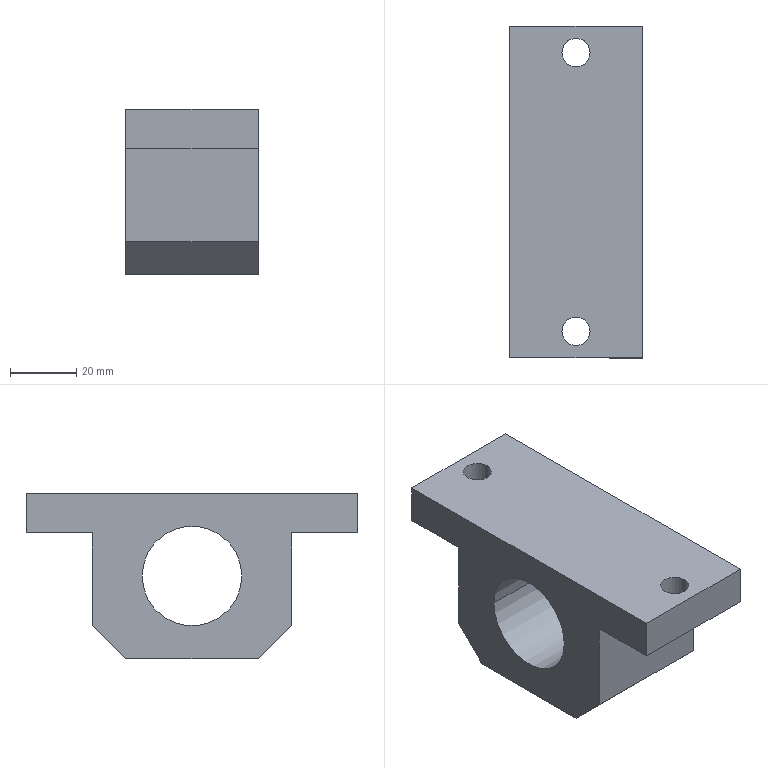Component | SolidWorks | AxisSeat-1 | 1 solid | 20 faces | box 40 x 100 x 50 mm | volume 105366 mm3 | plane 12 | cylinder 8 | commonest cylinder face diameters 8.5 x4 5 x2 30 x2
build123d program:
from build123d import *

# Parameters (mm, degrees)
SKETCH1_R              = 15
BOSS_EXTRUDE1_DEPTH    = 40
SKETCH2_R              = 4.25
CUT_EXTRUDE1_DEPTH     = 82.24
CHAMFER1_SIZE          = 10
M6_TAPPED_HOLE1_REACH  = 83.24
M6_TAPPED_HOLE1_BORE_R = 2.5


with BuildPart() as part:
    # Sketch1 → Boss-Extrude1 (new body)
    with BuildSketch(Plane.XY):
        Polygon((-50, 0), (-50, 12), (-30, 12), (-30, 50), (30, 50), (30, 12), (50, 12), (50, 0), align=None)
        with Locations((0, 25)):
            Circle(SKETCH1_R, mode=Mode.SUBTRACT)
    extrude(amount=BOSS_EXTRUDE1_DEPTH)

    # Sketch2 → Cut-Extrude1 (cut, through all)
    with BuildSketch(Plane.XZ):
        with Locations(Location((-42, 20, 0), (0, 0, 270))):
            Circle(SKETCH2_R)
        with Locations(Location((42, 20, 0), (0, 0, 270))):
            Circle(SKETCH2_R)
    extrude(amount=-CUT_EXTRUDE1_DEPTH, mode=Mode.SUBTRACT)

    # Chamfer1
    chamfer1_edges = [part.edges().sort_by_distance(p)[0] for p in [
        (-30, 50, 20),
        (30, 50, 20),
    ]]
    chamfer(chamfer1_edges, length=CHAMFER1_SIZE)

    # M6 Tapped Hole1 bore → M6 Tapped Hole1 (cut, up to next)
    with BuildSketch(Plane(origin=(0, 50, 0), x_dir=(1, 0, 0), z_dir=(0, 1, 0)), mode=Mode.PRIVATE) as m6_tapped_hole1_sk1:
        with Locations((0, -20)):
            Circle(M6_TAPPED_HOLE1_BORE_R)
    m6_tapped_hole1_tool1 = extrude(m6_tapped_hole1_sk1.sketch, amount=-M6_TAPPED_HOLE1_REACH, mode=Mode.PRIVATE) & part.part
    add(m6_tapped_hole1_tool1.solids().sort_by_distance((0, 50, 20))[0], mode=Mode.SUBTRACT)


solid = part.part

# Placed as in the assembly
solid = solid.moved(Location((894.468, -62.684, 1336.399), (-90, 90, 0)))
STEP:
#1=COLOUR_RGB('',0.7922,0.8196,0.9333);
#2=FILL_AREA_STYLE_COLOUR('',#1);
#3=FILL_AREA_STYLE('',(#2));
#4=SURFACE_STYLE_FILL_AREA(#3);
#5=SURFACE_SIDE_STYLE('',(#4));
#6=SURFACE_STYLE_USAGE(.BOTH.,#5);
#7=PRESENTATION_STYLE_ASSIGNMENT((#6));
#8=CARTESIAN_POINT('',(35.904,-2.468,51.039));
#9=VERTEX_POINT('',#8);
#10=CARTESIAN_POINT('',(36.101,-2.468,51.039));
#11=VERTEX_POINT('',#10);
#12=CARTESIAN_POINT('',(35.904,-2.468,51.039));
#13=CARTESIAN_POINT('',(35.904,-2.474,51.039));
#14=CARTESIAN_POINT('',(35.905,-2.481,51.039));
#15=CARTESIAN_POINT('',(35.907,-2.493,51.04));
#16=CARTESIAN_POINT('',(35.909,-2.5,51.04));
#17=CARTESIAN_POINT('',(35.914,-2.512,51.041));
#18=CARTESIAN_POINT('',(35.917,-2.517,51.041));
#19=CARTESIAN_POINT('',(35.924,-2.528,51.042));
#20=CARTESIAN_POINT('',(35.929,-2.533,51.043));
#21=CARTESIAN_POINT('',(35.942,-2.547,51.045));
#22=CARTESIAN_POINT('',(35.953,-2.554,51.046));
#23=CARTESIAN_POINT('',(35.971,-2.561,51.047));
#24=CARTESIAN_POINT('',(35.977,-2.563,51.047));
#25=CARTESIAN_POINT('',(35.99,-2.566,51.047));
#26=CARTESIAN_POINT('',(35.996,-2.566,51.048));
#27=CARTESIAN_POINT('',(36.009,-2.566,51.048));
#28=CARTESIAN_POINT('',(36.016,-2.566,51.047));
#29=CARTESIAN_POINT('',(36.028,-2.563,51.047));
#30=CARTESIAN_POINT('',(36.034,-2.561,51.047));
#31=CARTESIAN_POINT('',(36.046,-2.556,51.046));
#32=CARTESIAN_POINT('',(36.052,-2.553,51.046));
#33=CARTESIAN_POINT('',(36.063,-2.546,51.045));
#34=CARTESIAN_POINT('',(36.068,-2.542,51.044));
#35=CARTESIAN_POINT('',(36.077,-2.533,51.043));
#36=CARTESIAN_POINT('',(36.081,-2.528,51.042));
#37=CARTESIAN_POINT('',(36.088,-2.517,51.041));
#38=CARTESIAN_POINT('',(36.091,-2.512,51.041));
#39=CARTESIAN_POINT('',(36.096,-2.5,51.04));
#40=CARTESIAN_POINT('',(36.098,-2.493,51.04));
#41=CARTESIAN_POINT('',(36.1,-2.481,51.039));
#42=CARTESIAN_POINT('',(36.101,-2.474,51.039));
#43=CARTESIAN_POINT('',(36.101,-2.468,51.039));
#44=B_SPLINE_CURVE_WITH_KNOTS('',3,(#12,#13,#14,#15,#16,#17,#18,#19,#20,#21,#22,#23,#24,#25,#26,#27,#28,#29,#30,#31,#32,#33,#34,#35,#36,#37,#38,#39,#40,#41,#42,#43),.UNSPECIFIED.,.F.,.F.,(4,2,2,2,2,2,2,2,2,2,2,2,2,2,2,4),(0.,0.0004894,0.0009787,0.001468,0.001957,0.002936,0.003426,0.003915,0.004404,0.004894,0.005383,0.005872,0.006362,0.006851,0.00734,0.00783),.UNSPECIFIED.);
#45=EDGE_CURVE('',#9,#11,#44,.T.);
#46=ORIENTED_EDGE('',*,*,#45,.T.);
#47=CARTESIAN_POINT('',(36.101,-2.468,50.646));
#48=VERTEX_POINT('',#47);
#49=CARTESIAN_POINT('',(36.101,-2.468,50.646));
#50=DIRECTION('',(0.,0.,-1.));
#51=VECTOR('',#50,39.37);
#52=LINE('',#49,#51);
#53=EDGE_CURVE('',#11,#48,#52,.T.);
#54=ORIENTED_EDGE('',*,*,#53,.T.);
#55=CARTESIAN_POINT('',(35.904,-2.468,50.646));
#56=VERTEX_POINT('',#55);
#57=CARTESIAN_POINT('',(36.003,-2.468,50.646));
#58=DIRECTION('',(0.,0.,-1.));
#59=DIRECTION('',(-1.,0.,0.));
#60=AXIS2_PLACEMENT_3D('',#57,#58,#59);
#61=CIRCLE('',#60,0.09843);
#62=EDGE_CURVE('',#48,#56,#61,.T.);
#63=ORIENTED_EDGE('',*,*,#62,.T.);
#64=CARTESIAN_POINT('',(35.904,-2.468,50.646));
#65=DIRECTION('',(0.,0.,-1.));
#66=VECTOR('',#65,39.37);
#67=LINE('',#64,#66);
#68=EDGE_CURVE('',#9,#56,#67,.T.);
#69=ORIENTED_EDGE('',*,*,#68,.F.);
#70=EDGE_LOOP('',(#46,#54,#63,#69));
#71=FACE_OUTER_BOUND('',#70,.T.);
#72=CARTESIAN_POINT('',(36.003,-2.468,50.646));
#73=DIRECTION('',(0.,0.,-1.));
#74=DIRECTION('',(-1.,0.,0.));
#75=AXIS2_PLACEMENT_3D('',#72,#73,#74);
#76=CYLINDRICAL_SURFACE('',#75,0.09843);
#77=ADVANCED_FACE('',(#71),#76,.F.);
#78=CARTESIAN_POINT('',(35.835,-0.8143,52.142));
#79=VERTEX_POINT('',#78);
#80=CARTESIAN_POINT('',(36.17,-0.8143,52.142));
#81=VERTEX_POINT('',#80);
#82=CARTESIAN_POINT('',(36.003,-0.8143,52.142));
#83=DIRECTION('',(-0.,0.,1.));
#84=DIRECTION('',(0.,1.,0.));
#85=AXIS2_PLACEMENT_3D('',#82,#83,#84);
#86=CIRCLE('',#85,0.1673);
#87=EDGE_CURVE('',#79,#81,#86,.T.);
#88=ORIENTED_EDGE('',*,*,#87,.F.);
#89=CARTESIAN_POINT('',(35.835,-0.8143,52.614));
#90=VERTEX_POINT('',#89);
#91=CARTESIAN_POINT('',(35.835,-0.8143,50.646));
#92=DIRECTION('',(-0.,-0.,1.));
#93=VECTOR('',#92,39.37);
#94=LINE('',#91,#93);
#95=EDGE_CURVE('',#79,#90,#94,.T.);
#96=ORIENTED_EDGE('',*,*,#95,.T.);
#97=CARTESIAN_POINT('',(36.17,-0.8143,52.614));
#98=VERTEX_POINT('',#97);
#99=CARTESIAN_POINT('',(36.003,-0.8143,52.614));
#100=DIRECTION('',(-0.,-0.,1.));
#101=DIRECTION('',(1.,0.,0.));
#102=AXIS2_PLACEMENT_3D('',#99,#100,#101);
#103=CIRCLE('',#102,0.1673);
#104=EDGE_CURVE('',#90,#98,#103,.T.);
#105=ORIENTED_EDGE('',*,*,#104,.T.);
#106=CARTESIAN_POINT('',(36.17,-0.8143,50.646));
#107=DIRECTION('',(-0.,-0.,1.));
#108=VECTOR('',#107,39.37);
#109=LINE('',#106,#108);
#110=EDGE_CURVE('',#81,#98,#109,.T.);
#111=ORIENTED_EDGE('',*,*,#110,.F.);
#112=EDGE_LOOP('',(#88,#96,#105,#111));
#113=FACE_OUTER_BOUND('',#112,.T.);
#114=CARTESIAN_POINT('',(36.003,-0.8143,50.646));
#115=DIRECTION('',(-0.,-0.,1.));
#116=DIRECTION('',(1.,0.,0.));
#117=AXIS2_PLACEMENT_3D('',#114,#115,#116);
#118=CYLINDRICAL_SURFACE('',#117,0.1673);
#119=ADVANCED_FACE('',(#113),#118,.F.);
#120=CARTESIAN_POINT('',(35.835,-4.121,52.142));
#121=VERTEX_POINT('',#120);
#122=CARTESIAN_POINT('',(36.17,-4.121,52.142));
#123=VERTEX_POINT('',#122);
#124=CARTESIAN_POINT('',(36.003,-4.121,52.142));
#125=DIRECTION('',(-0.,-0.,1.));
#126=DIRECTION('',(1.,0.,0.));
#127=AXIS2_PLACEMENT_3D('',#124,#125,#126);
#128=CIRCLE('',#127,0.1673);
#129=EDGE_CURVE('',#121,#123,#128,.T.);
#130=ORIENTED_EDGE('',*,*,#129,.F.);
#131=CARTESIAN_POINT('',(35.835,-4.121,52.614));
#132=VERTEX_POINT('',#131);
#133=CARTESIAN_POINT('',(35.835,-4.121,50.646));
#134=DIRECTION('',(-0.,-0.,1.));
#135=VECTOR('',#134,39.37);
#136=LINE('',#133,#135);
#137=EDGE_CURVE('',#121,#132,#136,.T.);
#138=ORIENTED_EDGE('',*,*,#137,.T.);
#139=CARTESIAN_POINT('',(36.17,-4.121,52.614));
#140=VERTEX_POINT('',#139);
#141=CARTESIAN_POINT('',(36.003,-4.121,52.614));
#142=DIRECTION('',(-0.,-0.,1.));
#143=DIRECTION('',(1.,0.,0.));
#144=AXIS2_PLACEMENT_3D('',#141,#142,#143);
#145=CIRCLE('',#144,0.1673);
#146=EDGE_CURVE('',#132,#140,#145,.T.);
#147=ORIENTED_EDGE('',*,*,#146,.T.);
#148=CARTESIAN_POINT('',(36.17,-4.121,50.646));
#149=DIRECTION('',(-0.,-0.,1.));
#150=VECTOR('',#149,39.37);
#151=LINE('',#148,#150);
#152=EDGE_CURVE('',#123,#140,#151,.T.);
#153=ORIENTED_EDGE('',*,*,#152,.F.);
#154=EDGE_LOOP('',(#130,#138,#147,#153));
#155=FACE_OUTER_BOUND('',#154,.T.);
#156=CARTESIAN_POINT('',(36.003,-4.121,50.646));
#157=DIRECTION('',(-0.,-0.,1.));
#158=DIRECTION('',(1.,0.,0.));
#159=AXIS2_PLACEMENT_3D('',#156,#157,#158);
#160=CYLINDRICAL_SURFACE('',#159,0.1673);
#161=ADVANCED_FACE('',(#155),#160,.F.);
#162=CARTESIAN_POINT('',(35.215,-3.058,51.63));
#163=VERTEX_POINT('',#162);
#164=CARTESIAN_POINT('',(35.215,-1.877,51.63));
#165=VERTEX_POINT('',#164);
#166=CARTESIAN_POINT('',(35.215,-2.468,51.63));
#167=DIRECTION('',(-1.,0.,-0.));
#168=DIRECTION('',(0.,1.,0.));
#169=AXIS2_PLACEMENT_3D('',#166,#167,#168);
#170=CIRCLE('',#169,0.5906);
#171=EDGE_CURVE('',#163,#165,#170,.T.);
#172=ORIENTED_EDGE('',*,*,#171,.T.);
#173=CARTESIAN_POINT('',(36.79,-1.877,51.63));
#174=VERTEX_POINT('',#173);
#175=CARTESIAN_POINT('',(35.215,-1.877,51.63));
#176=DIRECTION('',(1.,-0.,0.));
#177=VECTOR('',#176,39.37);
#178=LINE('',#175,#177);
#179=EDGE_CURVE('',#165,#174,#178,.T.);
#180=ORIENTED_EDGE('',*,*,#179,.T.);
#181=CARTESIAN_POINT('',(36.79,-3.058,51.63));
#182=VERTEX_POINT('',#181);
#183=CARTESIAN_POINT('',(36.79,-2.468,51.63));
#184=DIRECTION('',(-1.,0.,-0.));
#185=DIRECTION('',(0.,1.,0.));
#186=AXIS2_PLACEMENT_3D('',#183,#184,#185);
#187=CIRCLE('',#186,0.5906);
#188=EDGE_CURVE('',#182,#174,#187,.T.);
#189=ORIENTED_EDGE('',*,*,#188,.F.);
#190=CARTESIAN_POINT('',(35.215,-3.058,51.63));
#191=DIRECTION('',(1.,-0.,0.));
#192=VECTOR('',#191,39.37);
#193=LINE('',#190,#192);
#194=EDGE_CURVE('',#163,#182,#193,.T.);
#195=ORIENTED_EDGE('',*,*,#194,.F.);
#196=EDGE_LOOP('',(#172,#180,#189,#195));
#197=FACE_OUTER_BOUND('',#196,.T.);
#198=CARTESIAN_POINT('',(35.215,-2.468,51.63));
#199=DIRECTION('',(1.,-0.,0.));
#200=DIRECTION('',(0.,-1.,0.));
#201=AXIS2_PLACEMENT_3D('',#198,#199,#200);
#202=CYLINDRICAL_SURFACE('',#201,0.5906);
#203=ADVANCED_FACE('',(#197),#202,.F.);
#204=CARTESIAN_POINT('',(35.215,-1.287,52.142));
#205=VERTEX_POINT('',#204);
#206=CARTESIAN_POINT('',(35.215,-1.287,51.039));
#207=VERTEX_POINT('',#206);
#208=CARTESIAN_POINT('',(35.215,-1.287,50.646));
#209=DIRECTION('',(0.,-0.,-1.));
#210=VECTOR('',#209,39.37);
#211=LINE('',#208,#210);
#212=EDGE_CURVE('',#205,#207,#211,.T.);
#213=ORIENTED_EDGE('',*,*,#212,.T.);
#214=CARTESIAN_POINT('',(35.215,-1.68,50.646));
#215=VERTEX_POINT('',#214);
#216=CARTESIAN_POINT('',(35.215,-1.09,51.236));
#217=DIRECTION('',(0.,-0.7071,-0.7071));
#218=VECTOR('',#217,39.37);
#219=LINE('',#216,#218);
#220=EDGE_CURVE('',#207,#215,#219,.T.);
#221=ORIENTED_EDGE('',*,*,#220,.T.);
#222=CARTESIAN_POINT('',(35.215,-3.255,50.646));
#223=VERTEX_POINT('',#222);
#224=CARTESIAN_POINT('',(35.215,-3.649,50.646));
#225=DIRECTION('',(-0.,-1.,-0.));
#226=VECTOR('',#225,39.37);
#227=LINE('',#224,#226);
#228=EDGE_CURVE('',#215,#223,#227,.T.);
#229=ORIENTED_EDGE('',*,*,#228,.T.);
#230=CARTESIAN_POINT('',(35.215,-3.649,51.039));
#231=VERTEX_POINT('',#230);
#232=CARTESIAN_POINT('',(35.215,-3.846,51.236));
#233=DIRECTION('',(-0.,-0.7071,0.7071));
#234=VECTOR('',#233,39.37);
#235=LINE('',#232,#234);
#236=EDGE_CURVE('',#223,#231,#235,.T.);
#237=ORIENTED_EDGE('',*,*,#236,.T.);
#238=CARTESIAN_POINT('',(35.215,-3.649,52.142));
#239=VERTEX_POINT('',#238);
#240=CARTESIAN_POINT('',(35.215,-3.649,50.646));
#241=DIRECTION('',(-0.,-0.,1.));
#242=VECTOR('',#241,39.37);
#243=LINE('',#240,#242);
#244=EDGE_CURVE('',#231,#239,#243,.T.);
#245=ORIENTED_EDGE('',*,*,#244,.T.);
#246=CARTESIAN_POINT('',(35.215,-4.436,52.142));
#247=VERTEX_POINT('',#246);
#248=CARTESIAN_POINT('',(35.215,-4.436,52.142));
#249=DIRECTION('',(-0.,-1.,-0.));
#250=VECTOR('',#249,39.37);
#251=LINE('',#248,#250);
#252=EDGE_CURVE('',#239,#247,#251,.T.);
#253=ORIENTED_EDGE('',*,*,#252,.T.);
#254=CARTESIAN_POINT('',(35.215,-4.436,52.614));
#255=VERTEX_POINT('',#254);
#256=CARTESIAN_POINT('',(35.215,-4.436,52.614));
#257=DIRECTION('',(-0.,-0.,1.));
#258=VECTOR('',#257,39.37);
#259=LINE('',#256,#258);
#260=EDGE_CURVE('',#247,#255,#259,.T.);
#261=ORIENTED_EDGE('',*,*,#260,.T.);
#262=CARTESIAN_POINT('',(35.215,-0.4994,52.614));
#263=VERTEX_POINT('',#262);
#264=CARTESIAN_POINT('',(35.215,-4.436,52.614));
#265=DIRECTION('',(0.,1.,0.));
#266=VECTOR('',#265,39.37);
#267=LINE('',#264,#266);
#268=EDGE_CURVE('',#255,#263,#267,.T.);
#269=ORIENTED_EDGE('',*,*,#268,.T.);
#270=CARTESIAN_POINT('',(35.215,-0.4994,52.142));
#271=VERTEX_POINT('',#270);
#272=CARTESIAN_POINT('',(35.215,-0.4994,52.614));
#273=DIRECTION('',(0.,0.,-1.));
#274=VECTOR('',#273,39.37);
#275=LINE('',#272,#274);
#276=EDGE_CURVE('',#263,#271,#275,.T.);
#277=ORIENTED_EDGE('',*,*,#276,.T.);
#278=CARTESIAN_POINT('',(35.215,-0.4994,52.142));
#279=DIRECTION('',(-0.,-1.,0.));
#280=VECTOR('',#279,39.37);
#281=LINE('',#278,#280);
#282=EDGE_CURVE('',#271,#205,#281,.T.);
#283=ORIENTED_EDGE('',*,*,#282,.T.);
#284=EDGE_LOOP('',(#213,#221,#229,#237,#245,#253,#261,#269,#277,#283));
#285=FACE_OUTER_BOUND('',#284,.T.);
#286=ORIENTED_EDGE('',*,*,#171,.F.);
#287=CARTESIAN_POINT('',(35.215,-2.468,51.63));
#288=DIRECTION('',(-1.,0.,-0.));
#289=DIRECTION('',(0.,1.,0.));
#290=AXIS2_PLACEMENT_3D('',#287,#288,#289);
#291=CIRCLE('',#290,0.5906);
#292=EDGE_CURVE('',#165,#163,#291,.T.);
#293=ORIENTED_EDGE('',*,*,#292,.F.);
#294=EDGE_LOOP('',(#286,#293));
#295=FACE_BOUND('',#294,.T.);
#296=CARTESIAN_POINT('',(35.215,-2.468,52.614));
#297=DIRECTION('',(-1.,0.,-0.));
#298=DIRECTION('',(0.,1.,0.));
#299=AXIS2_PLACEMENT_3D('',#296,#297,#298);
#300=PLANE('',#299);
#301=ADVANCED_FACE('',(#285,#295),#300,.T.);
#302=CARTESIAN_POINT('',(36.79,-1.68,50.646));
#303=VERTEX_POINT('',#302);
#304=CARTESIAN_POINT('',(36.79,-3.255,50.646));
#305=VERTEX_POINT('',#304);
#306=CARTESIAN_POINT('',(36.79,-3.649,50.646));
#307=DIRECTION('',(-0.,-1.,-0.));
#308=VECTOR('',#307,39.37);
#309=LINE('',#306,#308);
#310=EDGE_CURVE('',#303,#305,#309,.T.);
#311=ORIENTED_EDGE('',*,*,#310,.F.);
#312=CARTESIAN_POINT('',(36.79,-1.287,51.039));
#313=VERTEX_POINT('',#312);
#314=CARTESIAN_POINT('',(36.79,-1.68,50.646));
#315=DIRECTION('',(-0.,0.7071,0.7071));
#316=VECTOR('',#315,39.37);
#317=LINE('',#314,#316);
#318=EDGE_CURVE('',#303,#313,#317,.T.);
#319=ORIENTED_EDGE('',*,*,#318,.T.);
#320=CARTESIAN_POINT('',(36.79,-1.287,52.142));
#321=VERTEX_POINT('',#320);
#322=CARTESIAN_POINT('',(36.79,-1.287,50.646));
#323=DIRECTION('',(0.,-0.,-1.));
#324=VECTOR('',#323,39.37);
#325=LINE('',#322,#324);
#326=EDGE_CURVE('',#321,#313,#325,.T.);
#327=ORIENTED_EDGE('',*,*,#326,.F.);
#328=CARTESIAN_POINT('',(36.79,-0.4994,52.142));
#329=VERTEX_POINT('',#328);
#330=CARTESIAN_POINT('',(36.79,-0.4994,52.142));
#331=DIRECTION('',(-0.,-1.,0.));
#332=VECTOR('',#331,39.37);
#333=LINE('',#330,#332);
#334=EDGE_CURVE('',#329,#321,#333,.T.);
#335=ORIENTED_EDGE('',*,*,#334,.F.);
#336=CARTESIAN_POINT('',(36.79,-0.4994,52.614));
#337=VERTEX_POINT('',#336);
#338=CARTESIAN_POINT('',(36.79,-0.4994,52.614));
#339=DIRECTION('',(0.,0.,-1.));
#340=VECTOR('',#339,39.37);
#341=LINE('',#338,#340);
#342=EDGE_CURVE('',#337,#329,#341,.T.);
#343=ORIENTED_EDGE('',*,*,#342,.F.);
#344=CARTESIAN_POINT('',(36.79,-4.436,52.614));
#345=VERTEX_POINT('',#344);
#346=CARTESIAN_POINT('',(36.79,-4.436,52.614));
#347=DIRECTION('',(0.,1.,0.));
#348=VECTOR('',#347,39.37);
#349=LINE('',#346,#348);
#350=EDGE_CURVE('',#345,#337,#349,.T.);
#351=ORIENTED_EDGE('',*,*,#350,.F.);
#352=CARTESIAN_POINT('',(36.79,-4.436,52.142));
#353=VERTEX_POINT('',#352);
#354=CARTESIAN_POINT('',(36.79,-4.436,52.614));
#355=DIRECTION('',(-0.,-0.,1.));
#356=VECTOR('',#355,39.37);
#357=LINE('',#354,#356);
#358=EDGE_CURVE('',#353,#345,#357,.T.);
#359=ORIENTED_EDGE('',*,*,#358,.F.);
#360=CARTESIAN_POINT('',(36.79,-3.649,52.142));
#361=VERTEX_POINT('',#360);
#362=CARTESIAN_POINT('',(36.79,-4.436,52.142));
#363=DIRECTION('',(-0.,-1.,-0.));
#364=VECTOR('',#363,39.37);
#365=LINE('',#362,#364);
#366=EDGE_CURVE('',#361,#353,#365,.T.);
#367=ORIENTED_EDGE('',*,*,#366,.F.);
#368=CARTESIAN_POINT('',(36.79,-3.649,51.039));
#369=VERTEX_POINT('',#368);
#370=CARTESIAN_POINT('',(36.79,-3.649,50.646));
#371=DIRECTION('',(-0.,-0.,1.));
#372=VECTOR('',#371,39.37);
#373=LINE('',#370,#372);
#374=EDGE_CURVE('',#369,#361,#373,.T.);
#375=ORIENTED_EDGE('',*,*,#374,.F.);
#376=CARTESIAN_POINT('',(36.79,-3.649,51.039));
#377=DIRECTION('',(0.,0.7071,-0.7071));
#378=VECTOR('',#377,39.37);
#379=LINE('',#376,#378);
#380=EDGE_CURVE('',#369,#305,#379,.T.);
#381=ORIENTED_EDGE('',*,*,#380,.T.);
#382=EDGE_LOOP('',(#311,#319,#327,#335,#343,#351,#359,#367,#375,#381));
#383=FACE_OUTER_BOUND('',#382,.T.);
#384=ORIENTED_EDGE('',*,*,#188,.T.);
#385=CARTESIAN_POINT('',(36.79,-2.468,51.63));
#386=DIRECTION('',(-1.,0.,-0.));
#387=DIRECTION('',(0.,1.,0.));
#388=AXIS2_PLACEMENT_3D('',#385,#386,#387);
#389=CIRCLE('',#388,0.5906);
#390=EDGE_CURVE('',#174,#182,#389,.T.);
#391=ORIENTED_EDGE('',*,*,#390,.T.);
#392=EDGE_LOOP('',(#384,#391));
#393=FACE_BOUND('',#392,.T.);
#394=CARTESIAN_POINT('',(36.79,-2.468,52.614));
#395=DIRECTION('',(-1.,0.,-0.));
#396=DIRECTION('',(0.,1.,0.));
#397=AXIS2_PLACEMENT_3D('',#394,#395,#396);
#398=PLANE('',#397);
#399=ADVANCED_FACE('',(#383,#393),#398,.F.);
#400=CARTESIAN_POINT('',(36.003,-0.8143,52.614));
#401=DIRECTION('',(-0.,-0.,1.));
#402=DIRECTION('',(1.,0.,0.));
#403=AXIS2_PLACEMENT_3D('',#400,#401,#402);
#404=CIRCLE('',#403,0.1673);
#405=EDGE_CURVE('',#98,#90,#404,.T.);
#406=ORIENTED_EDGE('',*,*,#405,.F.);
#407=ORIENTED_EDGE('',*,*,#104,.F.);
#408=EDGE_LOOP('',(#406,#407));
#409=FACE_BOUND('',#408,.T.);
#410=CARTESIAN_POINT('',(36.003,-4.121,52.614));
#411=DIRECTION('',(-0.,-0.,1.));
#412=DIRECTION('',(1.,0.,0.));
#413=AXIS2_PLACEMENT_3D('',#410,#411,#412);
#414=CIRCLE('',#413,0.1673);
#415=EDGE_CURVE('',#140,#132,#414,.T.);
#416=ORIENTED_EDGE('',*,*,#415,.F.);
#417=ORIENTED_EDGE('',*,*,#146,.F.);
#418=EDGE_LOOP('',(#416,#417));
#419=FACE_BOUND('',#418,.T.);
#420=ORIENTED_EDGE('',*,*,#350,.T.);
#421=CARTESIAN_POINT('',(35.215,-0.4994,52.614));
#422=DIRECTION('',(1.,-0.,0.));
#423=VECTOR('',#422,39.37);
#424=LINE('',#421,#423);
#425=EDGE_CURVE('',#263,#337,#424,.T.);
#426=ORIENTED_EDGE('',*,*,#425,.F.);
#427=ORIENTED_EDGE('',*,*,#268,.F.);
#428=CARTESIAN_POINT('',(35.215,-4.436,52.614));
#429=DIRECTION('',(1.,-0.,0.));
#430=VECTOR('',#429,39.37);
#431=LINE('',#428,#430);
#432=EDGE_CURVE('',#255,#345,#431,.T.);
#433=ORIENTED_EDGE('',*,*,#432,.T.);
#434=EDGE_LOOP('',(#420,#426,#427,#433));
#435=FACE_OUTER_BOUND('',#434,.T.);
#436=CARTESIAN_POINT('',(35.215,-4.436,52.614));
#437=DIRECTION('',(0.,0.,-1.));
#438=DIRECTION('',(-1.,0.,-0.));
#439=AXIS2_PLACEMENT_3D('',#436,#437,#438);
#440=PLANE('',#439);
#441=ADVANCED_FACE('',(#409,#419,#435),#440,.F.);
#442=ORIENTED_EDGE('',*,*,#342,.T.);
#443=CARTESIAN_POINT('',(35.215,-0.4994,52.142));
#444=DIRECTION('',(1.,-0.,0.));
#445=VECTOR('',#444,39.37);
#446=LINE('',#443,#445);
#447=EDGE_CURVE('',#271,#329,#446,.T.);
#448=ORIENTED_EDGE('',*,*,#447,.F.);
#449=ORIENTED_EDGE('',*,*,#276,.F.);
#450=ORIENTED_EDGE('',*,*,#425,.T.);
#451=EDGE_LOOP('',(#442,#448,#449,#450));
#452=FACE_OUTER_BOUND('',#451,.T.);
#453=CARTESIAN_POINT('',(35.215,-0.4994,52.614));
#454=DIRECTION('',(-0.,-1.,-0.));
#455=DIRECTION('',(-1.,0.,-0.));
#456=AXIS2_PLACEMENT_3D('',#453,#454,#455);
#457=PLANE('',#456);
#458=ADVANCED_FACE('',(#452),#457,.F.);
#459=CARTESIAN_POINT('',(36.003,-0.8143,52.142));
#460=DIRECTION('',(-0.,0.,1.));
#461=DIRECTION('',(0.,1.,0.));
#462=AXIS2_PLACEMENT_3D('',#459,#460,#461);
#463=CIRCLE('',#462,0.1673);
#464=EDGE_CURVE('',#81,#79,#463,.T.);
#465=ORIENTED_EDGE('',*,*,#464,.T.);
#466=ORIENTED_EDGE('',*,*,#87,.T.);
#467=EDGE_LOOP('',(#465,#466));
#468=FACE_BOUND('',#467,.T.);
#469=ORIENTED_EDGE('',*,*,#334,.T.);
#470=CARTESIAN_POINT('',(35.215,-1.287,52.142));
#471=DIRECTION('',(1.,-0.,0.));
#472=VECTOR('',#471,39.37);
#473=LINE('',#470,#472);
#474=EDGE_CURVE('',#205,#321,#473,.T.);
#475=ORIENTED_EDGE('',*,*,#474,.F.);
#476=ORIENTED_EDGE('',*,*,#282,.F.);
#477=ORIENTED_EDGE('',*,*,#447,.T.);
#478=EDGE_LOOP('',(#469,#475,#476,#477));
#479=FACE_OUTER_BOUND('',#478,.T.);
#480=CARTESIAN_POINT('',(35.215,-0.4994,52.142));
#481=DIRECTION('',(-0.,0.,1.));
#482=DIRECTION('',(0.,1.,-0.));
#483=AXIS2_PLACEMENT_3D('',#480,#481,#482);
#484=PLANE('',#483);
#485=ADVANCED_FACE('',(#468,#479),#484,.F.);
#486=ORIENTED_EDGE('',*,*,#326,.T.);
#487=CARTESIAN_POINT('',(35.215,-1.287,51.039));
#488=DIRECTION('',(-1.,0.,-0.));
#489=VECTOR('',#488,39.37);
#490=LINE('',#487,#489);
#491=EDGE_CURVE('',#313,#207,#490,.T.);
#492=ORIENTED_EDGE('',*,*,#491,.T.);
#493=ORIENTED_EDGE('',*,*,#212,.F.);
#494=ORIENTED_EDGE('',*,*,#474,.T.);
#495=EDGE_LOOP('',(#486,#492,#493,#494));
#496=FACE_OUTER_BOUND('',#495,.T.);
#497=CARTESIAN_POINT('',(35.215,-1.287,50.646));
#498=DIRECTION('',(-0.,-1.,0.));
#499=DIRECTION('',(-0.,0.,1.));
#500=AXIS2_PLACEMENT_3D('',#497,#498,#499);
#501=PLANE('',#500);
#502=ADVANCED_FACE('',(#496),#501,.F.);
#503=CARTESIAN_POINT('',(36.003,-2.468,50.646));
#504=DIRECTION('',(0.,0.,-1.));
#505=DIRECTION('',(-1.,0.,0.));
#506=AXIS2_PLACEMENT_3D('',#503,#504,#505);
#507=CIRCLE('',#506,0.09843);
#508=EDGE_CURVE('',#56,#48,#507,.T.);
#509=ORIENTED_EDGE('',*,*,#508,.F.);
#510=ORIENTED_EDGE('',*,*,#62,.F.);
#511=EDGE_LOOP('',(#509,#510));
#512=FACE_BOUND('',#511,.T.);
#513=ORIENTED_EDGE('',*,*,#228,.F.);
#514=CARTESIAN_POINT('',(35.215,-1.68,50.646));
#515=DIRECTION('',(1.,-0.,0.));
#516=VECTOR('',#515,39.37);
#517=LINE('',#514,#516);
#518=EDGE_CURVE('',#215,#303,#517,.T.);
#519=ORIENTED_EDGE('',*,*,#518,.T.);
#520=ORIENTED_EDGE('',*,*,#310,.T.);
#521=CARTESIAN_POINT('',(35.215,-3.255,50.646));
#522=DIRECTION('',(-1.,0.,-0.));
#523=VECTOR('',#522,39.37);
#524=LINE('',#521,#523);
#525=EDGE_CURVE('',#305,#223,#524,.T.);
#526=ORIENTED_EDGE('',*,*,#525,.T.);
#527=EDGE_LOOP('',(#513,#519,#520,#526));
#528=FACE_OUTER_BOUND('',#527,.T.);
#529=CARTESIAN_POINT('',(35.215,-3.649,50.646));
#530=DIRECTION('',(-0.,-0.,1.));
#531=DIRECTION('',(0.,1.,0.));
#532=AXIS2_PLACEMENT_3D('',#529,#530,#531);
#533=PLANE('',#532);
#534=ADVANCED_FACE('',(#512,#528),#533,.F.);
#535=ORIENTED_EDGE('',*,*,#244,.F.);
#536=CARTESIAN_POINT('',(35.215,-3.649,51.039));
#537=DIRECTION('',(1.,-0.,0.));
#538=VECTOR('',#537,39.37);
#539=LINE('',#536,#538);
#540=EDGE_CURVE('',#231,#369,#539,.T.);
#541=ORIENTED_EDGE('',*,*,#540,.T.);
#542=ORIENTED_EDGE('',*,*,#374,.T.);
#543=CARTESIAN_POINT('',(35.215,-3.649,52.142));
#544=DIRECTION('',(1.,-0.,0.));
#545=VECTOR('',#544,39.37);
#546=LINE('',#543,#545);
#547=EDGE_CURVE('',#239,#361,#546,.T.);
#548=ORIENTED_EDGE('',*,*,#547,.F.);
#549=EDGE_LOOP('',(#535,#541,#542,#548));
#550=FACE_OUTER_BOUND('',#549,.T.);
#551=CARTESIAN_POINT('',(35.215,-3.649,50.646));
#552=DIRECTION('',(0.,1.,0.));
#553=DIRECTION('',(1.,-0.,0.));
#554=AXIS2_PLACEMENT_3D('',#551,#552,#553);
#555=PLANE('',#554);
#556=ADVANCED_FACE('',(#550),#555,.F.);
#557=CARTESIAN_POINT('',(36.003,-4.121,52.142));
#558=DIRECTION('',(-0.,-0.,1.));
#559=DIRECTION('',(1.,0.,0.));
#560=AXIS2_PLACEMENT_3D('',#557,#558,#559);
#561=CIRCLE('',#560,0.1673);
#562=EDGE_CURVE('',#123,#121,#561,.T.);
#563=ORIENTED_EDGE('',*,*,#562,.T.);
#564=ORIENTED_EDGE('',*,*,#129,.T.);
#565=EDGE_LOOP('',(#563,#564));
#566=FACE_BOUND('',#565,.T.);
#567=ORIENTED_EDGE('',*,*,#366,.T.);
#568=CARTESIAN_POINT('',(35.215,-4.436,52.142));
#569=DIRECTION('',(1.,-0.,0.));
#570=VECTOR('',#569,39.37);
#571=LINE('',#568,#570);
#572=EDGE_CURVE('',#247,#353,#571,.T.);
#573=ORIENTED_EDGE('',*,*,#572,.F.);
#574=ORIENTED_EDGE('',*,*,#252,.F.);
#575=ORIENTED_EDGE('',*,*,#547,.T.);
#576=EDGE_LOOP('',(#567,#573,#574,#575));
#577=FACE_OUTER_BOUND('',#576,.T.);
#578=CARTESIAN_POINT('',(35.215,-4.436,52.142));
#579=DIRECTION('',(-0.,-0.,1.));
#580=DIRECTION('',(1.,-0.,0.));
#581=AXIS2_PLACEMENT_3D('',#578,#579,#580);
#582=PLANE('',#581);
#583=ADVANCED_FACE('',(#566,#577),#582,.F.);
#584=ORIENTED_EDGE('',*,*,#358,.T.);
#585=ORIENTED_EDGE('',*,*,#432,.F.);
#586=ORIENTED_EDGE('',*,*,#260,.F.);
#587=ORIENTED_EDGE('',*,*,#572,.T.);
#588=EDGE_LOOP('',(#584,#585,#586,#587));
#589=FACE_OUTER_BOUND('',#588,.T.);
#590=CARTESIAN_POINT('',(35.215,-4.436,52.614));
#591=DIRECTION('',(0.,1.,0.));
#592=DIRECTION('',(1.,-0.,0.));
#593=AXIS2_PLACEMENT_3D('',#590,#591,#592);
#594=PLANE('',#593);
#595=ADVANCED_FACE('',(#589),#594,.F.);
#596=ORIENTED_EDGE('',*,*,#179,.F.);
#597=ORIENTED_EDGE('',*,*,#292,.T.);
#598=ORIENTED_EDGE('',*,*,#194,.T.);
#599=ORIENTED_EDGE('',*,*,#390,.F.);
#600=EDGE_LOOP('',(#596,#597,#598,#599));
#601=FACE_OUTER_BOUND('',#600,.T.);
#602=ORIENTED_EDGE('',*,*,#45,.F.);
#603=CARTESIAN_POINT('',(36.101,-2.468,51.039));
#604=CARTESIAN_POINT('',(36.101,-2.455,51.039));
#605=CARTESIAN_POINT('',(36.099,-2.442,51.04));
#606=CARTESIAN_POINT('',(36.091,-2.424,51.041));
#607=CARTESIAN_POINT('',(36.088,-2.419,51.041));
#608=CARTESIAN_POINT('',(36.081,-2.408,51.042));
#609=CARTESIAN_POINT('',(36.077,-2.403,51.043));
#610=CARTESIAN_POINT('',(36.068,-2.394,51.044));
#611=CARTESIAN_POINT('',(36.063,-2.39,51.045));
#612=CARTESIAN_POINT('',(36.052,-2.383,51.046));
#613=CARTESIAN_POINT('',(36.046,-2.379,51.046));
#614=CARTESIAN_POINT('',(36.035,-2.375,51.047));
#615=CARTESIAN_POINT('',(36.028,-2.373,51.047));
#616=CARTESIAN_POINT('',(36.016,-2.37,51.047));
#617=CARTESIAN_POINT('',(36.009,-2.369,51.048));
#618=CARTESIAN_POINT('',(35.996,-2.369,51.048));
#619=CARTESIAN_POINT('',(35.99,-2.37,51.047));
#620=CARTESIAN_POINT('',(35.977,-2.373,51.047));
#621=CARTESIAN_POINT('',(35.971,-2.374,51.047));
#622=CARTESIAN_POINT('',(35.959,-2.379,51.046));
#623=CARTESIAN_POINT('',(35.953,-2.382,51.046));
#624=CARTESIAN_POINT('',(35.943,-2.39,51.045));
#625=CARTESIAN_POINT('',(35.938,-2.394,51.044));
#626=CARTESIAN_POINT('',(35.924,-2.407,51.042));
#627=CARTESIAN_POINT('',(35.917,-2.418,51.041));
#628=CARTESIAN_POINT('',(35.909,-2.436,51.04));
#629=CARTESIAN_POINT('',(35.907,-2.442,51.04));
#630=CARTESIAN_POINT('',(35.905,-2.455,51.039));
#631=CARTESIAN_POINT('',(35.904,-2.461,51.039));
#632=CARTESIAN_POINT('',(35.904,-2.468,51.039));
#633=B_SPLINE_CURVE_WITH_KNOTS('',3,(#603,#604,#605,#606,#607,#608,#609,#610,#611,#612,#613,#614,#615,#616,#617,#618,#619,#620,#621,#622,#623,#624,#625,#626,#627,#628,#629,#630,#631,#632),.UNSPECIFIED.,.F.,.F.,(4,2,2,2,2,2,2,2,2,2,2,2,2,2,4),(0.00783,0.008808,0.009298,0.009787,0.01028,0.01077,0.01125,0.01174,0.01223,0.01272,0.01321,0.0137,0.01468,0.01517,0.01566),.UNSPECIFIED.);
#634=EDGE_CURVE('',#11,#9,#633,.T.);
#635=ORIENTED_EDGE('',*,*,#634,.F.);
#636=EDGE_LOOP('',(#602,#635));
#637=FACE_BOUND('',#636,.T.);
#638=CARTESIAN_POINT('',(35.215,-2.468,51.63));
#639=DIRECTION('',(1.,-0.,0.));
#640=DIRECTION('',(0.,-1.,0.));
#641=AXIS2_PLACEMENT_3D('',#638,#639,#640);
#642=CYLINDRICAL_SURFACE('',#641,0.5906);
#643=ADVANCED_FACE('',(#601,#637),#642,.F.);
#644=ORIENTED_EDGE('',*,*,#137,.F.);
#645=ORIENTED_EDGE('',*,*,#562,.F.);
#646=ORIENTED_EDGE('',*,*,#152,.T.);
#647=ORIENTED_EDGE('',*,*,#415,.T.);
#648=EDGE_LOOP('',(#644,#645,#646,#647));
#649=FACE_OUTER_BOUND('',#648,.T.);
#650=CARTESIAN_POINT('',(36.003,-4.121,50.646));
#651=DIRECTION('',(-0.,-0.,1.));
#652=DIRECTION('',(1.,0.,0.));
#653=AXIS2_PLACEMENT_3D('',#650,#651,#652);
#654=CYLINDRICAL_SURFACE('',#653,0.1673);
#655=ADVANCED_FACE('',(#649),#654,.F.);
#656=ORIENTED_EDGE('',*,*,#95,.F.);
#657=ORIENTED_EDGE('',*,*,#464,.F.);
#658=ORIENTED_EDGE('',*,*,#110,.T.);
#659=ORIENTED_EDGE('',*,*,#405,.T.);
#660=EDGE_LOOP('',(#656,#657,#658,#659));
#661=FACE_OUTER_BOUND('',#660,.T.);
#662=CARTESIAN_POINT('',(36.003,-0.8143,50.646));
#663=DIRECTION('',(-0.,-0.,1.));
#664=DIRECTION('',(1.,0.,0.));
#665=AXIS2_PLACEMENT_3D('',#662,#663,#664);
#666=CYLINDRICAL_SURFACE('',#665,0.1673);
#667=ADVANCED_FACE('',(#661),#666,.F.);
#668=ORIENTED_EDGE('',*,*,#220,.F.);
#669=ORIENTED_EDGE('',*,*,#491,.F.);
#670=ORIENTED_EDGE('',*,*,#318,.F.);
#671=ORIENTED_EDGE('',*,*,#518,.F.);
#672=EDGE_LOOP('',(#668,#669,#670,#671));
#673=FACE_OUTER_BOUND('',#672,.T.);
#674=CARTESIAN_POINT('',(35.215,-1.68,50.646));
#675=DIRECTION('',(-0.,-0.7071,0.7071));
#676=DIRECTION('',(1.,-0.,0.));
#677=AXIS2_PLACEMENT_3D('',#674,#675,#676);
#678=PLANE('',#677);
#679=ADVANCED_FACE('',(#673),#678,.F.);
#680=ORIENTED_EDGE('',*,*,#236,.F.);
#681=ORIENTED_EDGE('',*,*,#525,.F.);
#682=ORIENTED_EDGE('',*,*,#380,.F.);
#683=ORIENTED_EDGE('',*,*,#540,.F.);
#684=EDGE_LOOP('',(#680,#681,#682,#683));
#685=FACE_OUTER_BOUND('',#684,.T.);
#686=CARTESIAN_POINT('',(35.215,-3.649,51.039));
#687=DIRECTION('',(-0.,0.7071,0.7071));
#688=DIRECTION('',(1.,-0.,0.));
#689=AXIS2_PLACEMENT_3D('',#686,#687,#688);
#690=PLANE('',#689);
#691=ADVANCED_FACE('',(#685),#690,.F.);
#692=ORIENTED_EDGE('',*,*,#53,.F.);
#693=ORIENTED_EDGE('',*,*,#634,.T.);
#694=ORIENTED_EDGE('',*,*,#68,.T.);
#695=ORIENTED_EDGE('',*,*,#508,.T.);
#696=EDGE_LOOP('',(#692,#693,#694,#695));
#697=FACE_OUTER_BOUND('',#696,.T.);
#698=CARTESIAN_POINT('',(36.003,-2.468,50.646));
#699=DIRECTION('',(0.,0.,-1.));
#700=DIRECTION('',(-1.,0.,0.));
#701=AXIS2_PLACEMENT_3D('',#698,#699,#700);
#702=CYLINDRICAL_SURFACE('',#701,0.09843);
#703=ADVANCED_FACE('',(#697),#702,.F.);
#704=CLOSED_SHELL('',(#77,#119,#161,#203,#301,#399,#441,#458,#485,#502,#534,#556,#583,#595,#643,#655,#667,#679,#691,#703));
#705=MANIFOLD_SOLID_BREP('',#704);
#706=STYLED_ITEM('',(#7),#705);
#707=(LENGTH_UNIT()NAMED_UNIT(*)SI_UNIT($,.METRE.));
#708=LENGTH_MEASURE_WITH_UNIT(LENGTH_MEASURE(0.0254),#707);
#709=DIMENSIONAL_EXPONENTS(1.,0.,0.,0.,0.,0.,0.);
#710=(CONVERSION_BASED_UNIT('',#708)LENGTH_UNIT()NAMED_UNIT(#709));
#711=UNCERTAINTY_MEASURE_WITH_UNIT(LENGTH_MEASURE(0.00001),#710,'','');
#712=(NAMED_UNIT(*)PLANE_ANGLE_UNIT()SI_UNIT($,.RADIAN.));
#713=(NAMED_UNIT(*)SI_UNIT($,.STERADIAN.)SOLID_ANGLE_UNIT());
#714=(GEOMETRIC_REPRESENTATION_CONTEXT(3)GLOBAL_UNCERTAINTY_ASSIGNED_CONTEXT((#711))GLOBAL_UNIT_ASSIGNED_CONTEXT((#710,#712,#713))REPRESENTATION_CONTEXT('',''));
#715=MECHANICAL_DESIGN_GEOMETRIC_PRESENTATION_REPRESENTATION('',(#706),#714);
#716=CARTESIAN_POINT('',(0.,0.,0.));
#717=DIRECTION('',(0.,0.,1.));
#718=DIRECTION('',(1.,0.,0.));
#719=AXIS2_PLACEMENT_3D('',#716,#717,#718);
#720=(LENGTH_UNIT()NAMED_UNIT(*)SI_UNIT($,.METRE.));
#721=LENGTH_MEASURE_WITH_UNIT(LENGTH_MEASURE(0.0254),#720);
#722=DIMENSIONAL_EXPONENTS(1.,0.,0.,0.,0.,0.,0.);
#723=(CONVERSION_BASED_UNIT('',#721)LENGTH_UNIT()NAMED_UNIT(#722));
#724=UNCERTAINTY_MEASURE_WITH_UNIT(LENGTH_MEASURE(0.00001),#723,'','');
#725=(NAMED_UNIT(*)PLANE_ANGLE_UNIT()SI_UNIT($,.RADIAN.));
#726=(NAMED_UNIT(*)SI_UNIT($,.STERADIAN.)SOLID_ANGLE_UNIT());
#727=(GEOMETRIC_REPRESENTATION_CONTEXT(3)GLOBAL_UNCERTAINTY_ASSIGNED_CONTEXT((#724))GLOBAL_UNIT_ASSIGNED_CONTEXT((#723,#725,#726))REPRESENTATION_CONTEXT('',''));
#728=ADVANCED_BREP_SHAPE_REPRESENTATION('',(#705,#719),#727);
#729=PRESENTATION_LAYER_ASSIGNMENT('','',(#706));